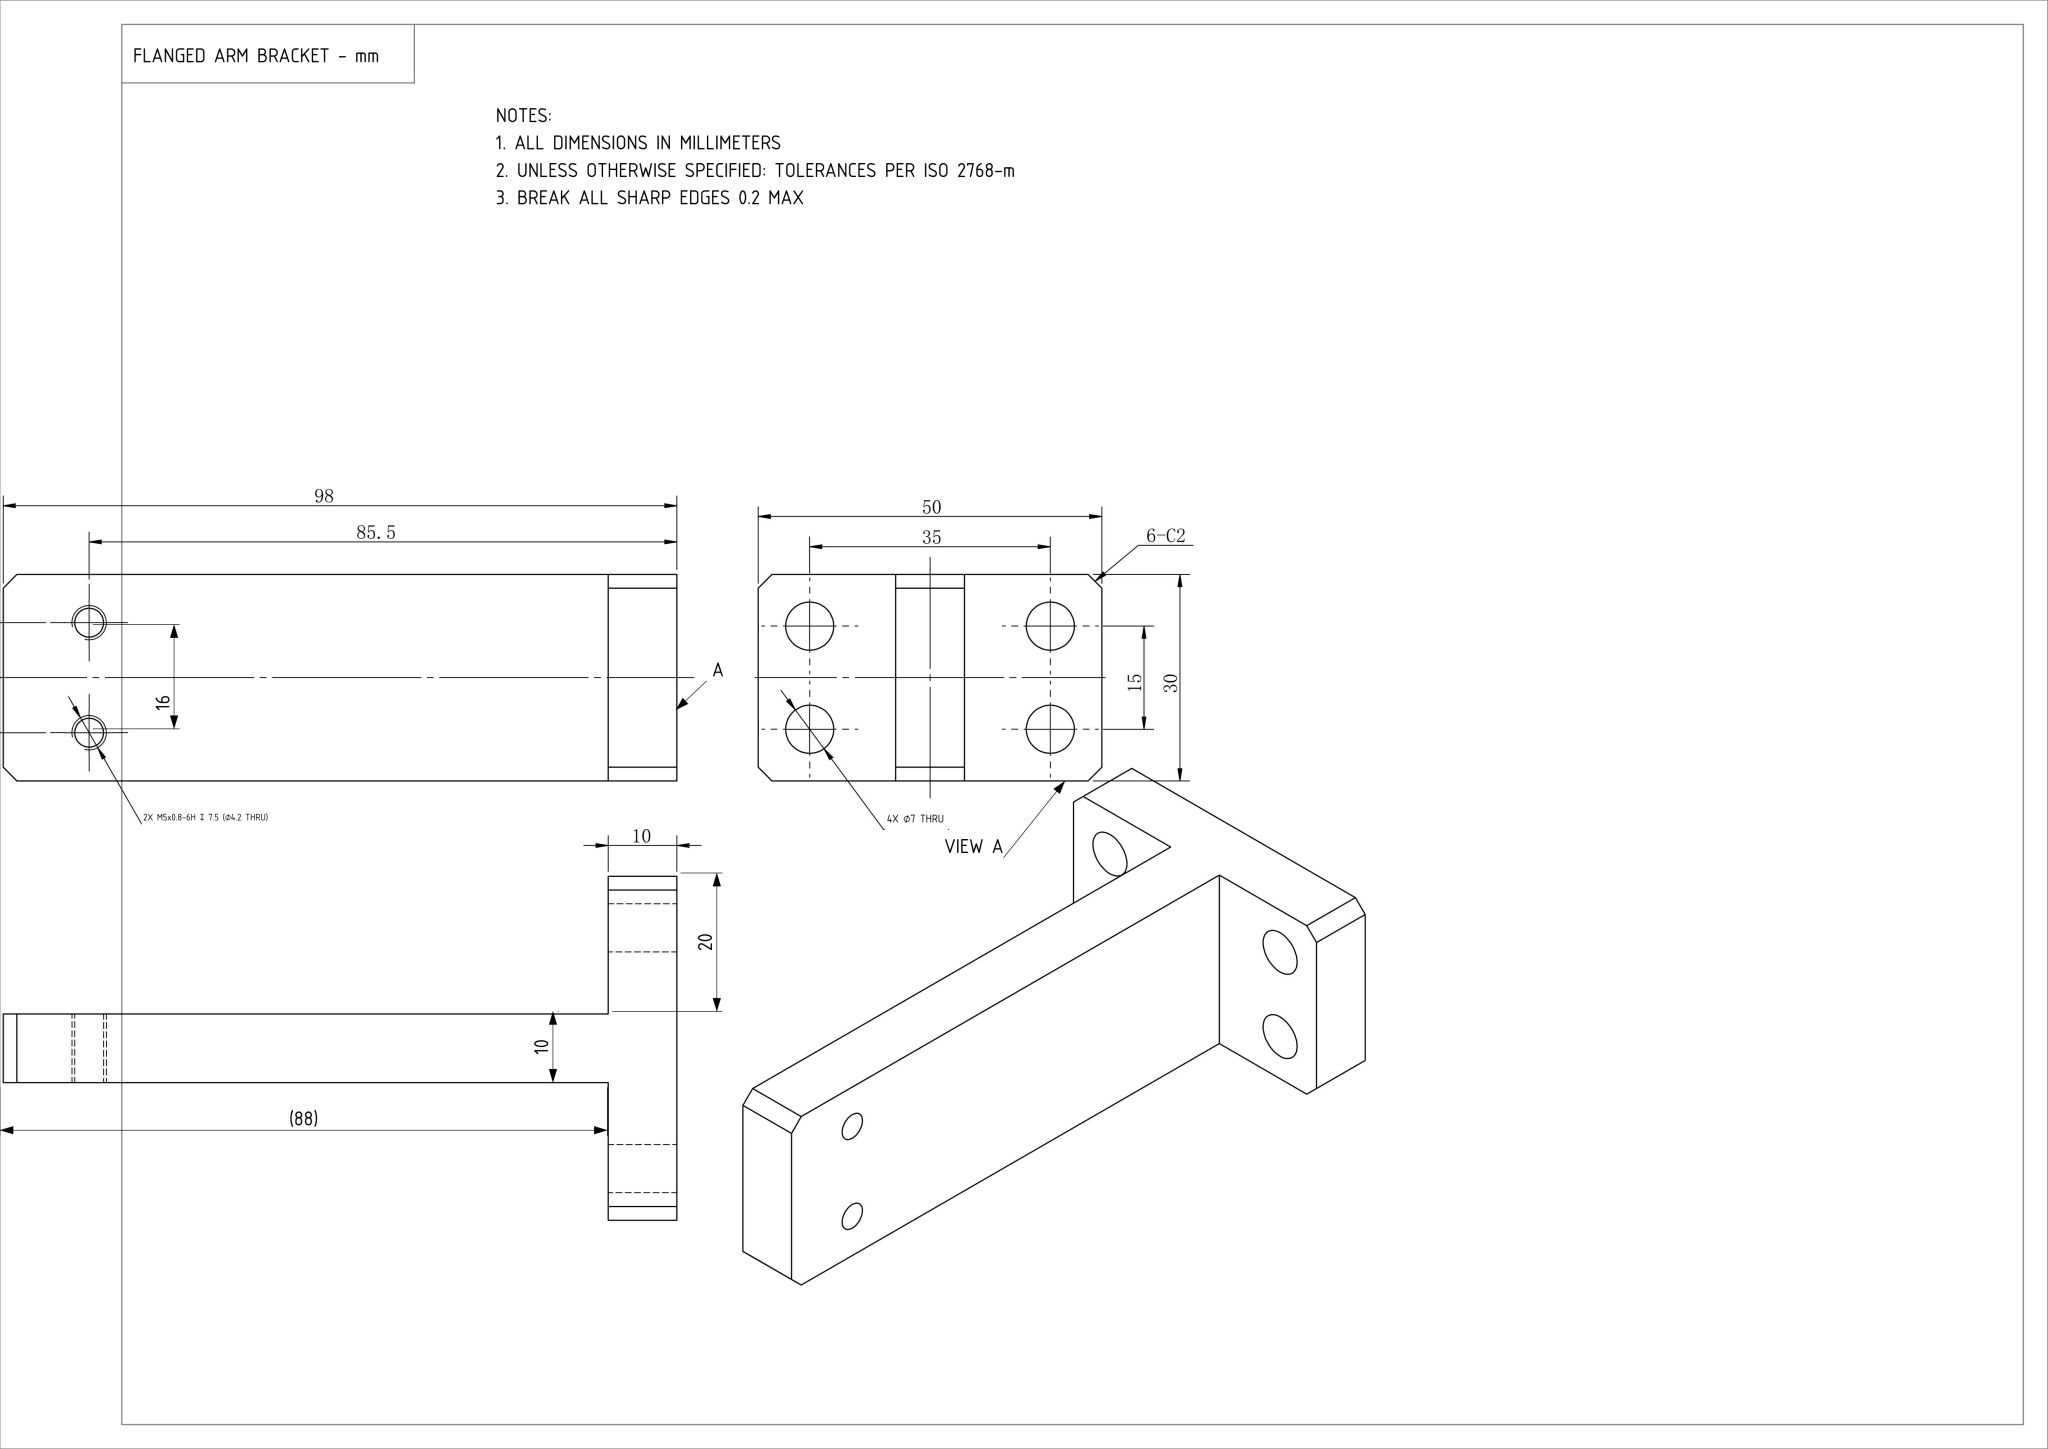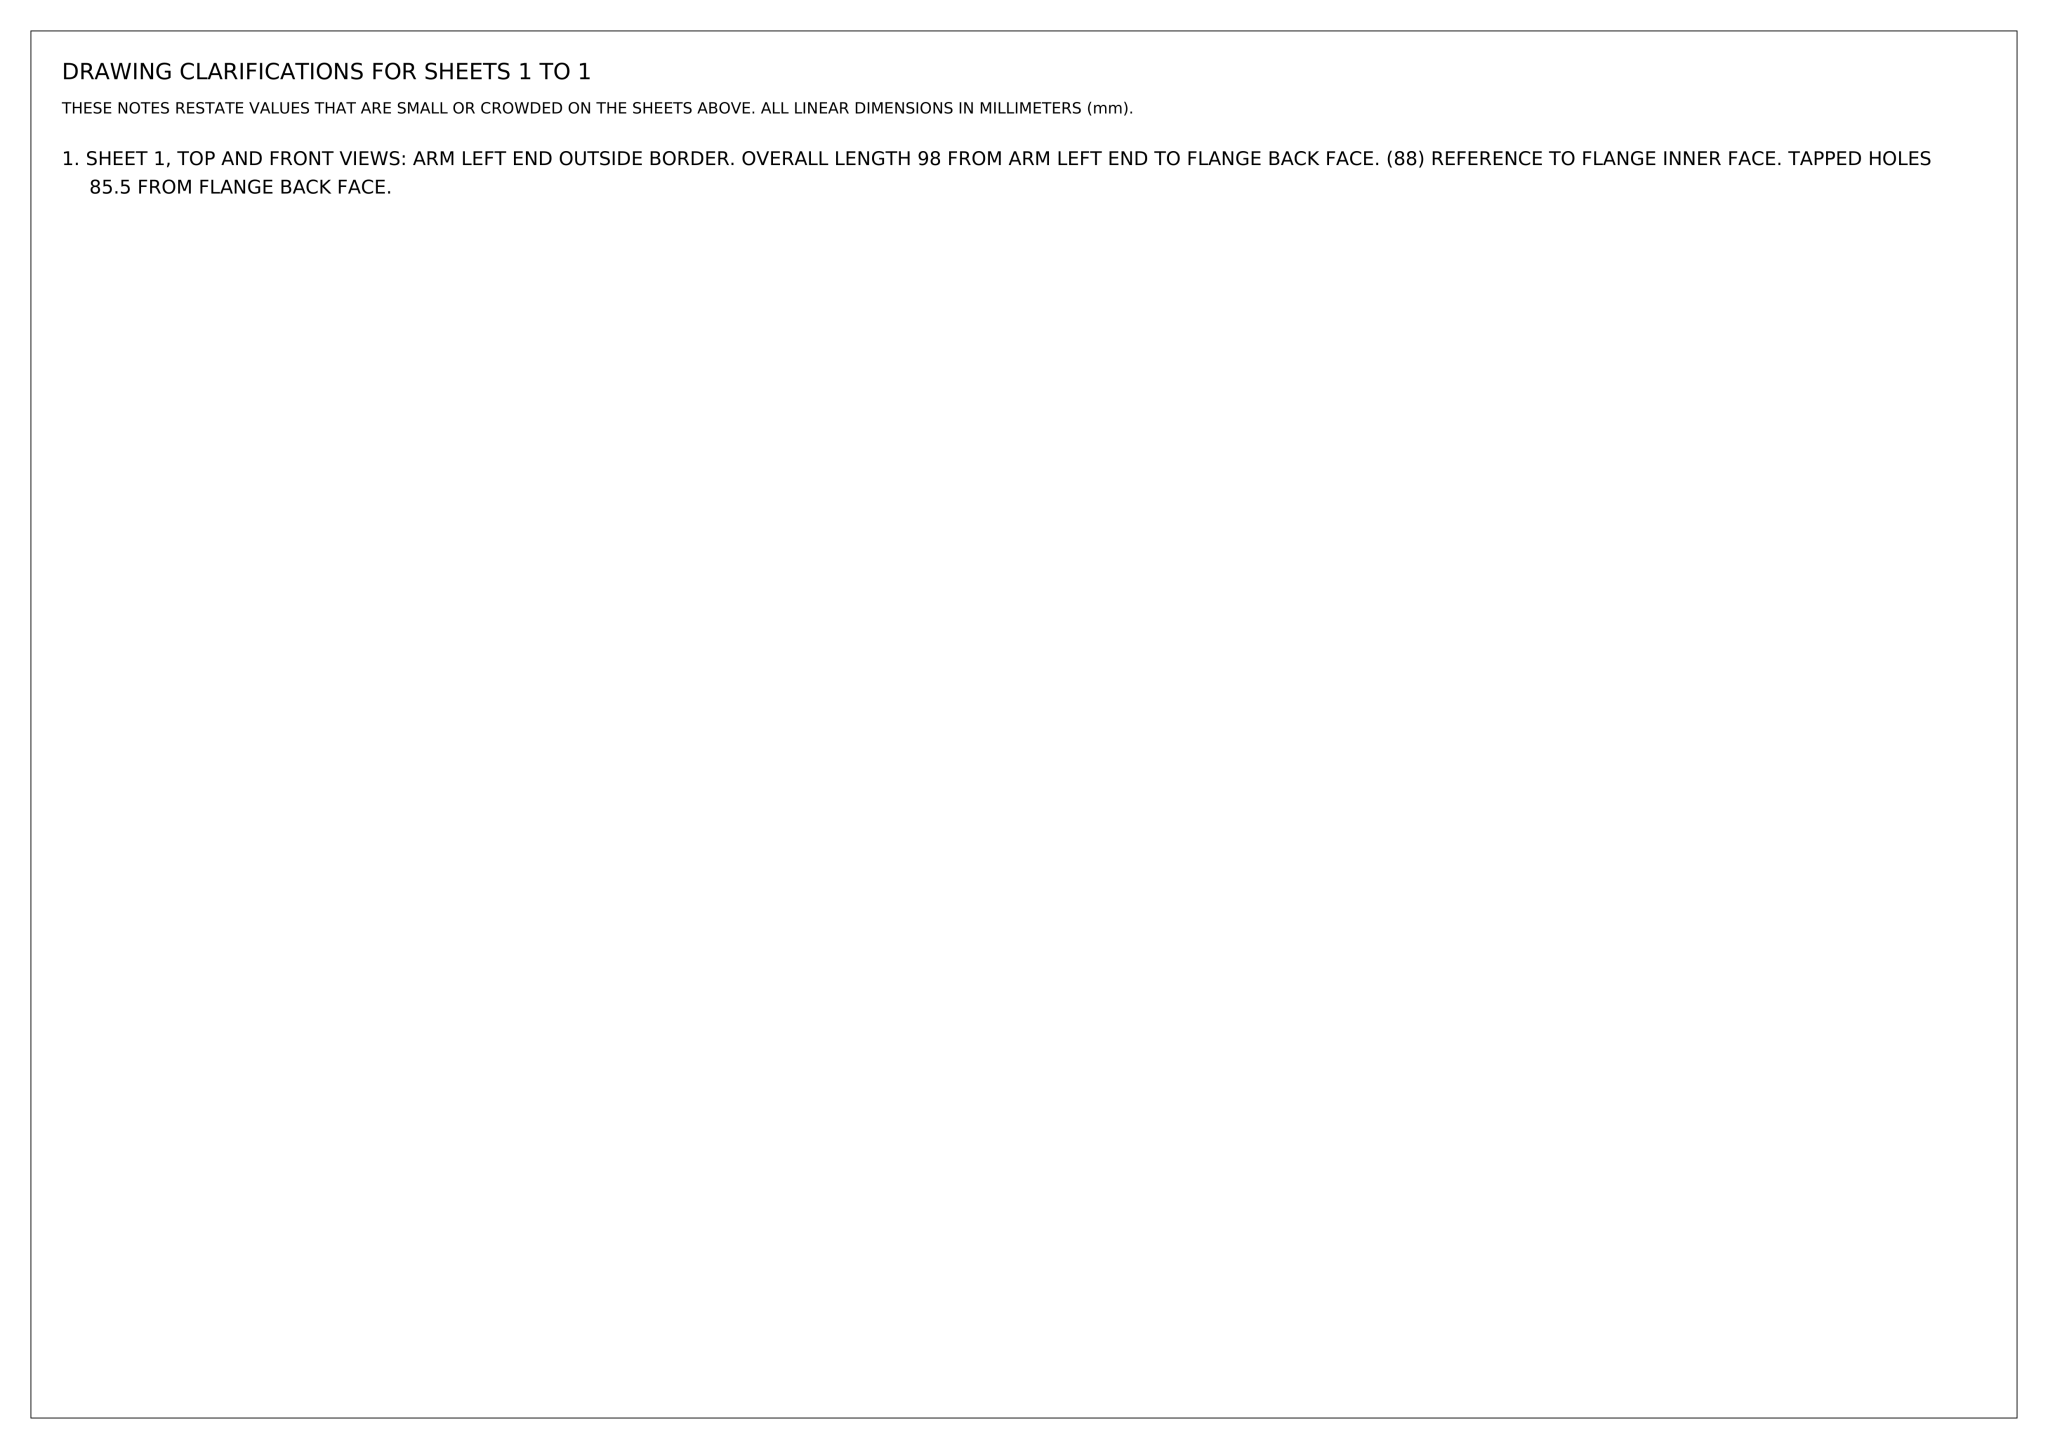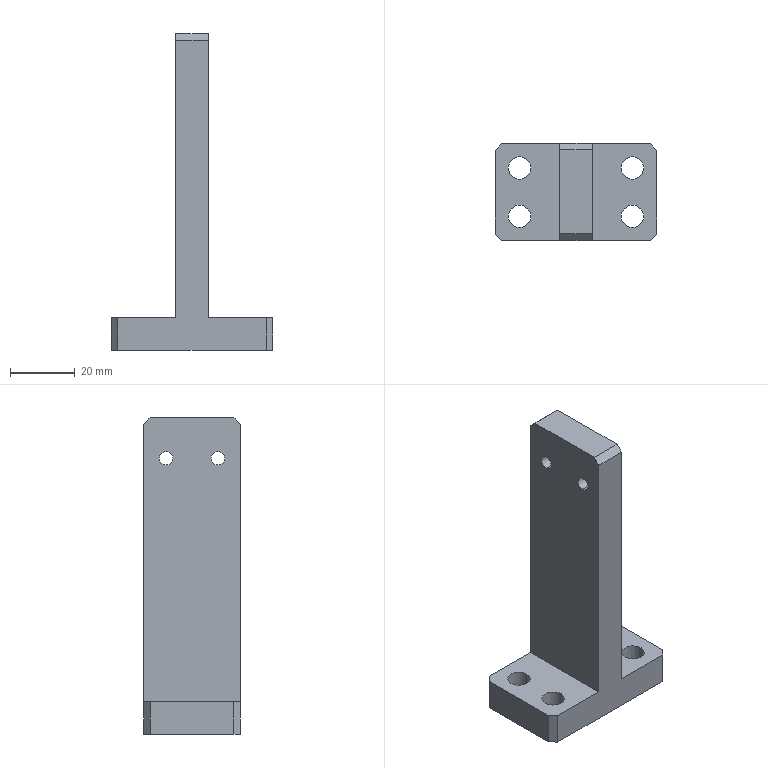Part | NX | mm | 1 solid | 28 faces | box 50 x 30 x 98 mm | volume 39464 mm3 | plane 16 | cylinder 12 | commonest cylinder face diameters 7 x8 4.2 x4